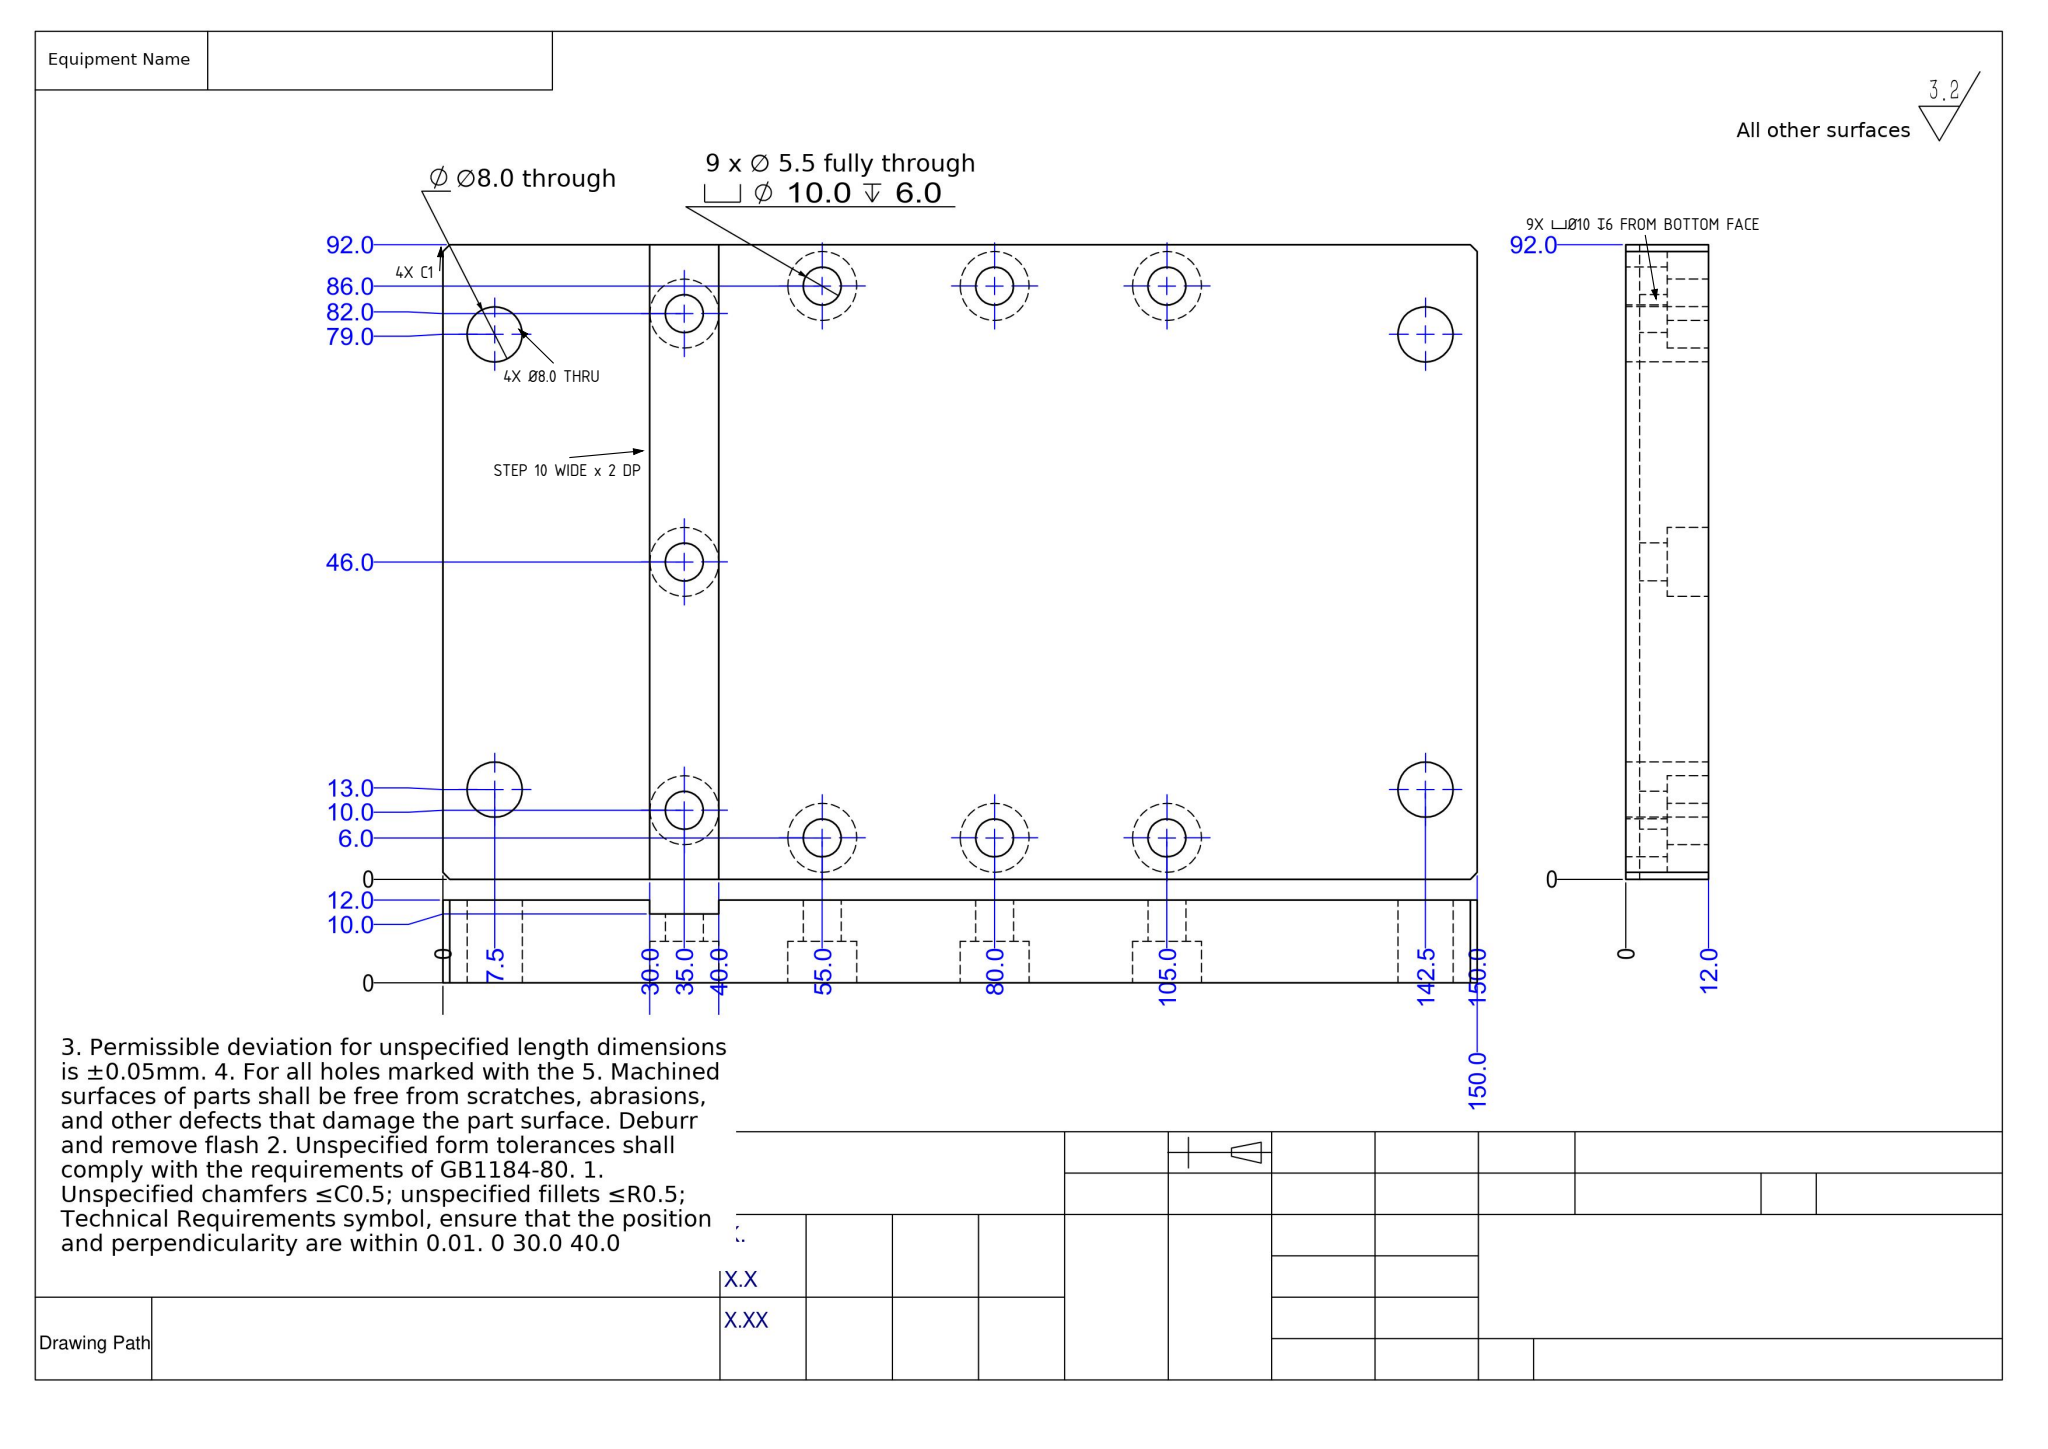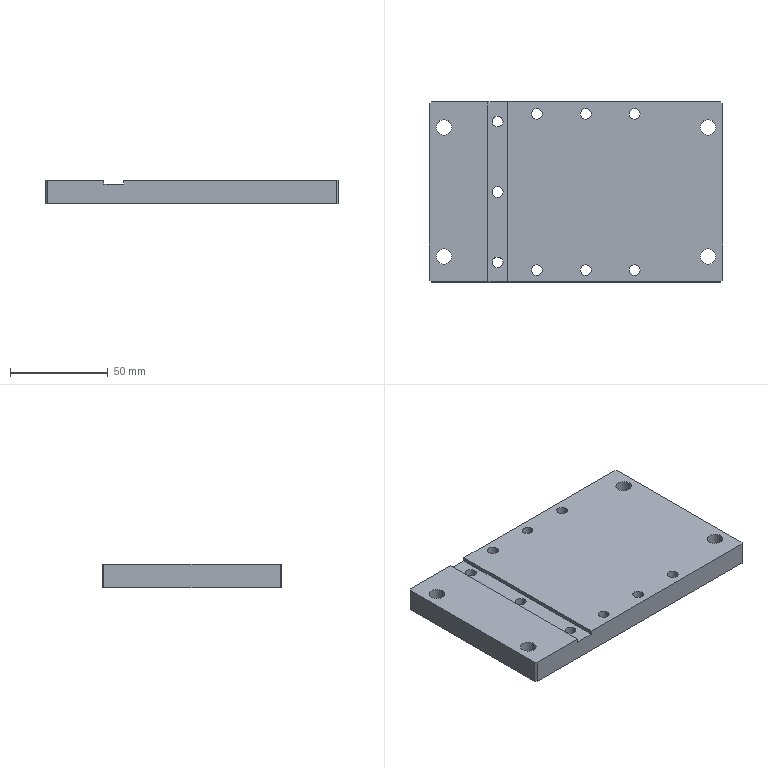Part | SolidWorks | mm | 1 solid | 67 faces | box 150 x 92 x 12 mm | volume 155942 mm3 | cylinder 44 | plane 23 | commonest cylinder face diameters 10 x18 5.5 x18 8 x8
Drawing notes:
STEP X30-X40: 10 WIDE x 2 DP FROM TOP FACE, FULL 92 HT | from the solid: x-planes at 30.0 & 40.0 (10 wide); z-plane 10.0 vs 12.0 top face => 2 deep; y-planes 0 & 92 full height
4X Ø8.0 THRU (12.0 THK), AT X=7.5 & X=142.5 FROM LEFT EDGE, Y=13.0 & Y=79.0 FROM BOTTOM EDGE | from the solid: cylinders [8.0,"z",[7.5,13.0]], [8.0,"z",[7.5,79.0]], [8.0,"z",[142.5,13.0]], [8.0,"z",[142.5,79.0]], length 12.0 = bbox Z 12.0
4X CHAMFER C1 AT CORNERS, FULL 12 THK | from the solid: 4 inclined planes 45°, size 1.0 x 1.0 x 12.0 at corners (0,0),(0,91),(149,0),(149,91)
9X C'BORE Ø10 DP 6 FROM BOTTOM FACE (0 IN SIDE VIEW) | from the solid: Ø10 bores run z=0 to 6; Ø5.5 continues to z=10/12; c'bore flats at z=6
build123d program:
from build123d import *

# Parameters (mm, degrees)
SKETCH1_W                                  = 150
SKETCH1_H                                  = 92
BOSS_EXTRUDE1_DEPTH                        = 12
SKETCH2_R                                  = 4
CUT_EXTRUDE1_DEPTH                         = 12
SKETCH4_W                                  = 10
SKETCH4_H                                  = 92
CUT_EXTRUDE3_DEPTH                         = 2
M5_HEX_HEAD_BOLT_COUNTERBORE_1_D           = 5.5
M5_HEX_HEAD_BOLT_COUNTERBORE_1_CBORE_D     = 10
M5_HEX_HEAD_BOLT_COUNTERBORE_1_CBORE_DEPTH = 6
CHAMFER1_SIZE                              = 1


with BuildPart() as part:
    # Sketch1 → Boss-Extrude1 (new body)
    with BuildSketch(Plane.XY):
        Rectangle(SKETCH1_W, SKETCH1_H)
    extrude(amount=BOSS_EXTRUDE1_DEPTH)

    # Sketch2 → Cut-Extrude1 (cut)
    with BuildSketch(Plane.XY.offset(12)):
        with Locations((-67.5, 33)):
            Circle(SKETCH2_R)
        with Locations(Location((-67.5, -33, 0), (0, 0, 180))):
            Circle(SKETCH2_R)
        with Locations((67.5, -33)):
            Circle(SKETCH2_R)
        with Locations(Location((67.5, 33, 0), (0, 0, 180))):
            Circle(SKETCH2_R)
    extrude(amount=-CUT_EXTRUDE1_DEPTH, mode=Mode.SUBTRACT)

    # Sketch4 → Cut-Extrude3 (cut)
    with BuildSketch(Plane.XY.offset(12)):
        with Locations((-40, 0)):
            Rectangle(SKETCH4_W, SKETCH4_H)
    extrude(amount=-CUT_EXTRUDE3_DEPTH, mode=Mode.SUBTRACT)

    # M5 Hex head bolt counterbore 1 (through all)
    with Locations(Plane(origin=(0, 0, 0), x_dir=(-1, 0, 0), z_dir=(0, 0, -1))):
        with Locations((40, -36), (40, 0), (40, 36), (20, -40), (20, 40), (-5, 40), (-30, 40), (-30, -40), (-5, -40)):
            CounterBoreHole(M5_HEX_HEAD_BOLT_COUNTERBORE_1_D / 2, M5_HEX_HEAD_BOLT_COUNTERBORE_1_CBORE_D / 2, M5_HEX_HEAD_BOLT_COUNTERBORE_1_CBORE_DEPTH)

    # Chamfer1
    chamfer1_edges = [part.edges().sort_by_distance(p)[0] for p in [
        (75, -46, 6),
        (-75, -46, 6),
        (-75, 46, 6),
        (75, 46, 6),
    ]]
    chamfer(chamfer1_edges, length=CHAMFER1_SIZE)


solid = part.part